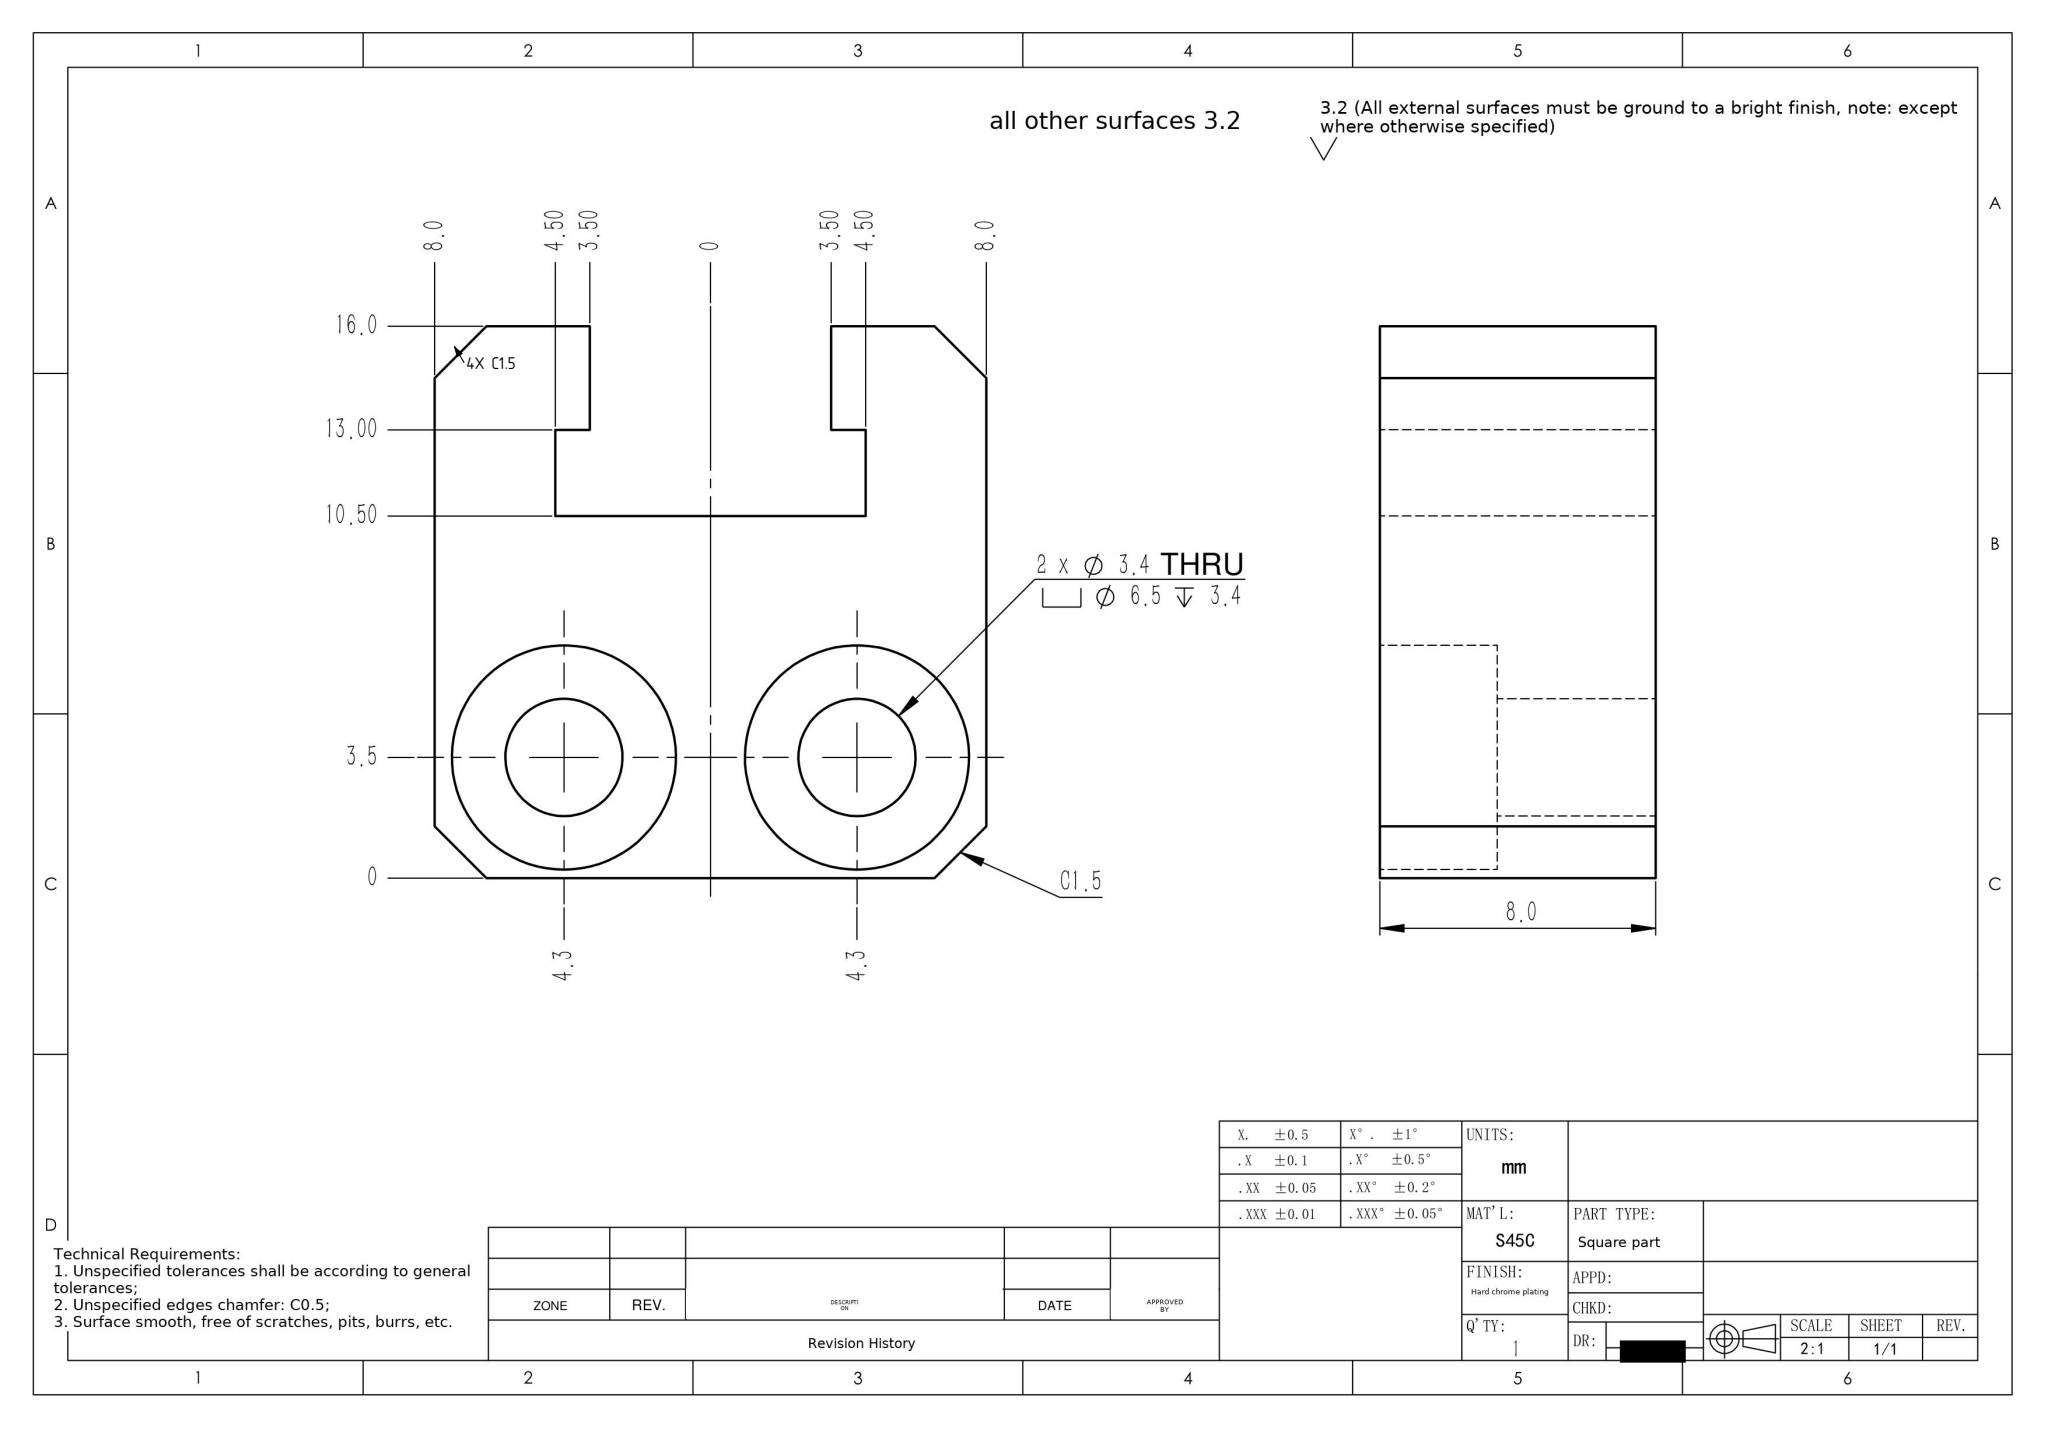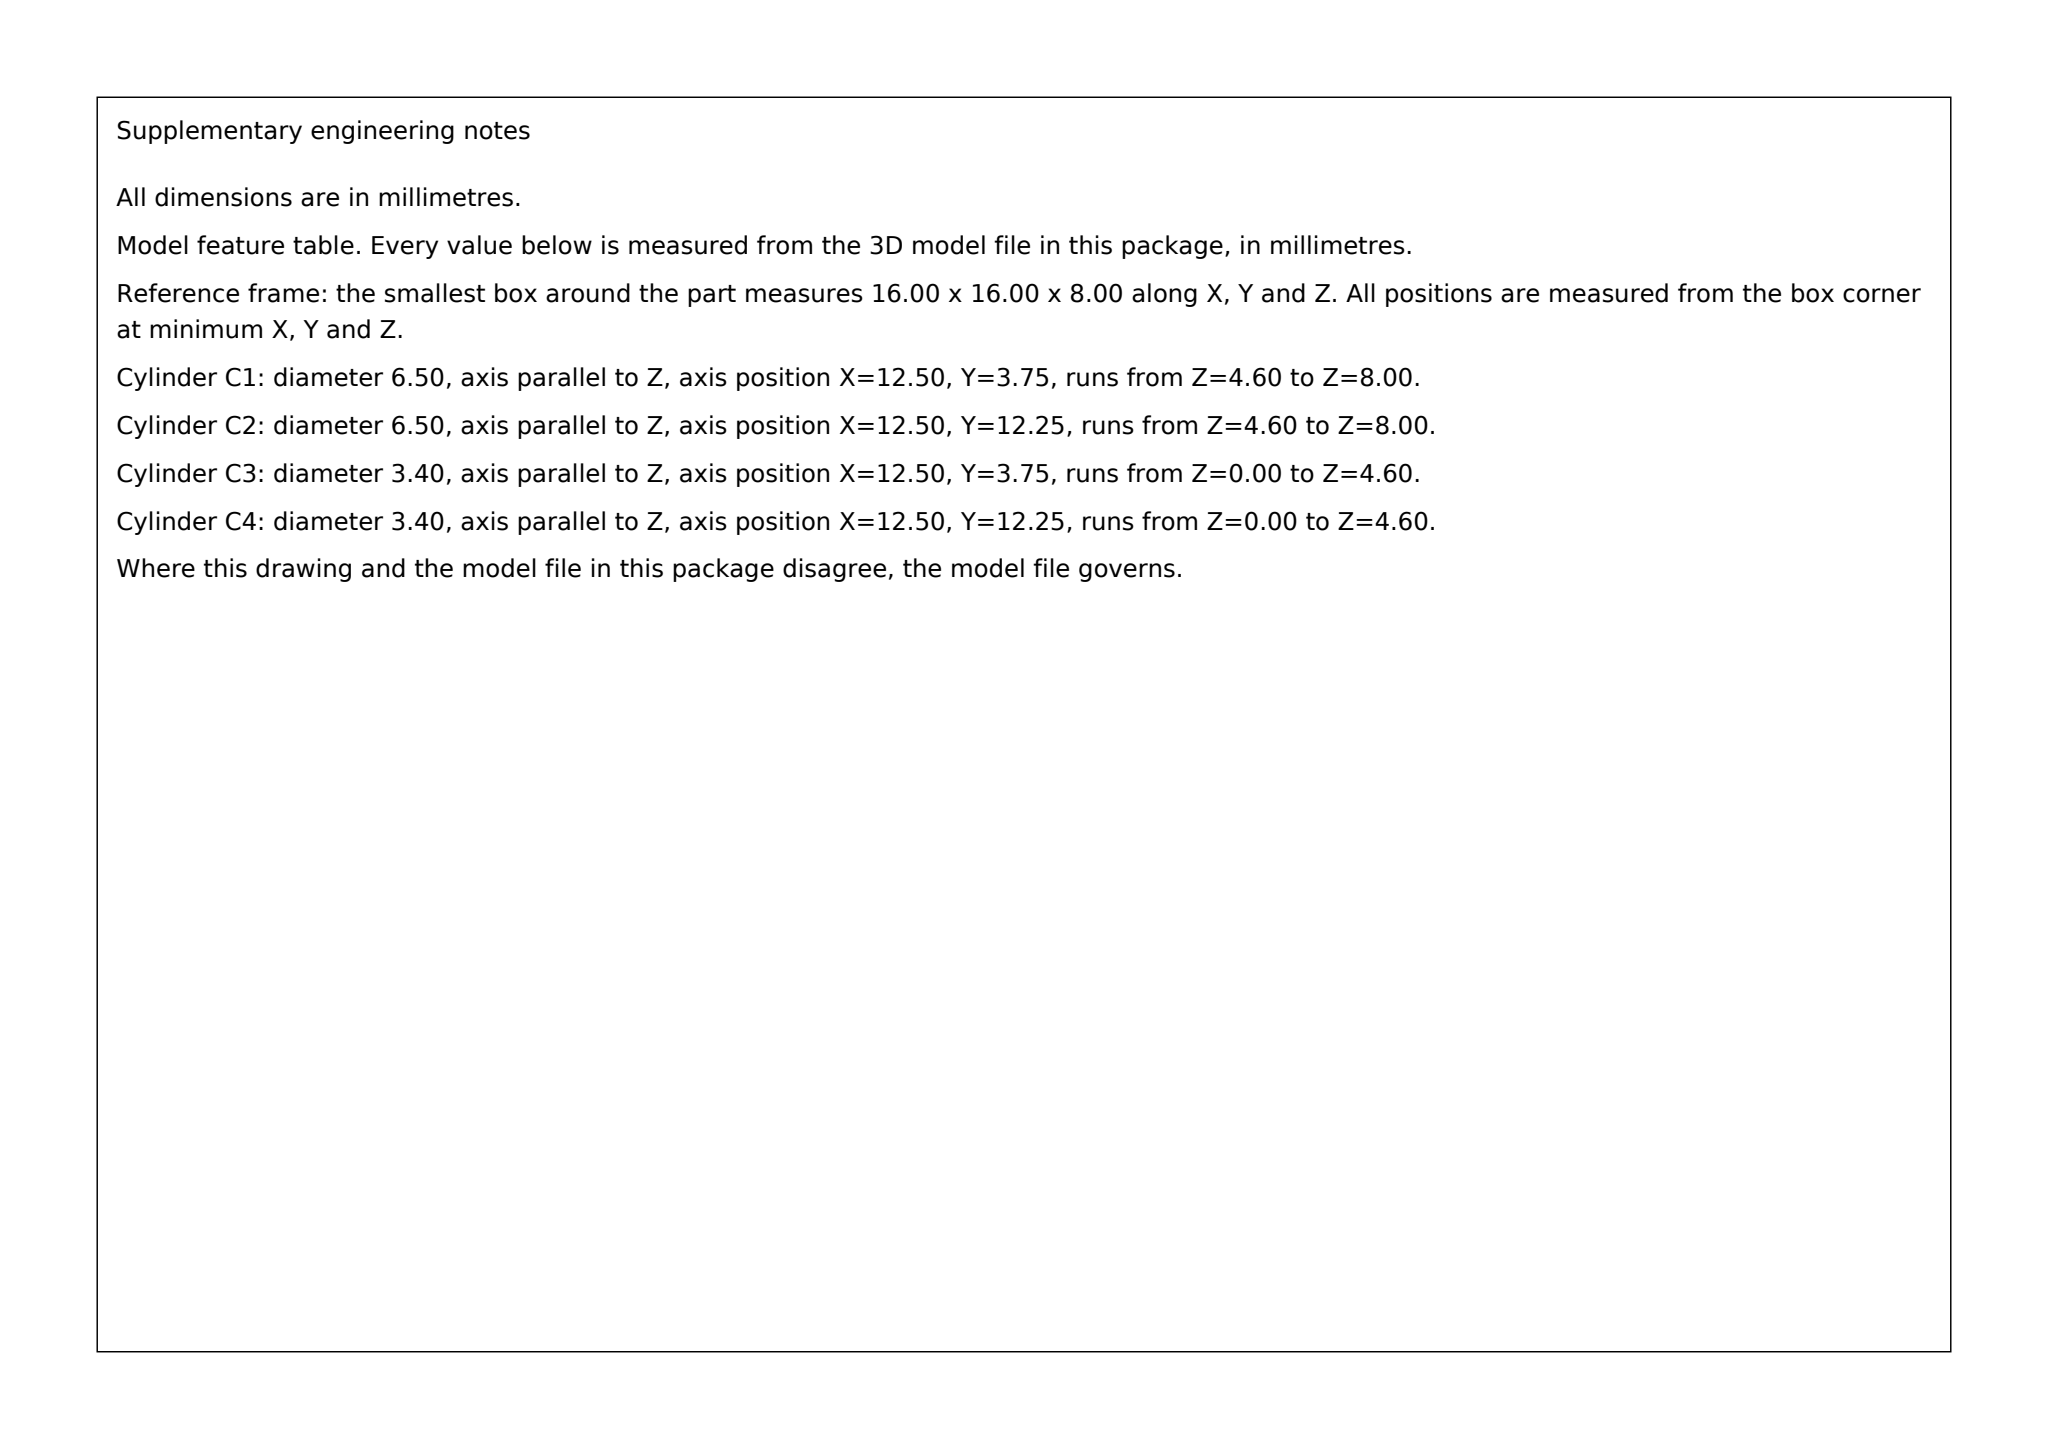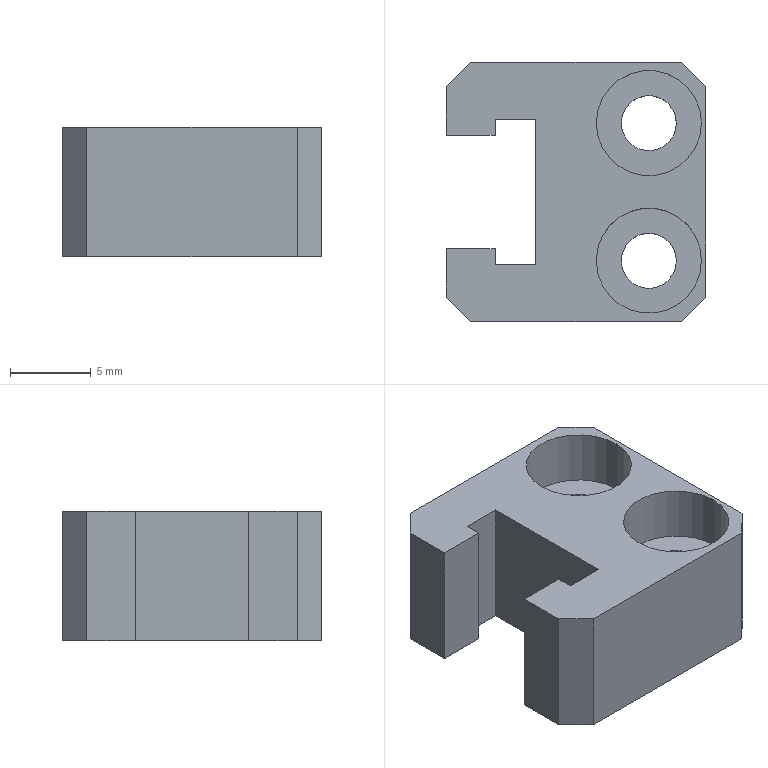Part | SolidWorks | mm | material S45C | 1 solid | 28 faces | box 16 x 16 x 8 mm | volume 1355 mm3 | plane 20 | cylinder 8 | commonest cylinder face diameters 6.5 x4 3.4 x4
Drawing notes:
4X C1.5 x 45° AT CORNERS OF 16 x 16 OUTLINE | from the solid: Bbox 16x16x8; outline bounded by planes x=0/16, y=0/16; all four outline corners broken equally, matching existing C1.5 callout (part symmetric about y=8 centerline)
build123d program:
from build123d import *

# Parameters (mm, degrees)
SKETCH1_W                                       = 16
SKETCH1_H                                       = 16
BOSS_EXTRUDE1_DEPTH                             = 8
M3_HEX_SOCKET_HEAD_CAP_SCREW_CBORE1_D           = 3.4
M3_HEX_SOCKET_HEAD_CAP_SCREW_CBORE1_CBORE_D     = 6.5
M3_HEX_SOCKET_HEAD_CAP_SCREW_CBORE1_CBORE_DEPTH = 3.4
CUT_EXTRUDE1_DEPTH                              = 20.596
CHAMFER1_SIZE                                   = 1.5


with BuildPart() as part:
    # Sketch1 → Boss-Extrude1 (new body)
    with BuildSketch(Plane.XY):
        with Locations((8, 0)):
            Rectangle(SKETCH1_W, SKETCH1_H)
    extrude(amount=BOSS_EXTRUDE1_DEPTH)

    # M3 Hex Socket Head Cap Screw CBORE1 (through all)
    with Locations(Plane.XY.offset(8)):
        with Locations((12.5, 4.25), (12.5, -4.25)):
            CounterBoreHole(M3_HEX_SOCKET_HEAD_CAP_SCREW_CBORE1_D / 2, M3_HEX_SOCKET_HEAD_CAP_SCREW_CBORE1_CBORE_D / 2, M3_HEX_SOCKET_HEAD_CAP_SCREW_CBORE1_CBORE_DEPTH)

    # Sketch4 → Cut-Extrude1 (cut, through all)
    with BuildSketch(Plane.XY.offset(8)):
        Polygon((0, -3.5), (0, 3.5), (3, 3.5), (3, 4.5), (5.5, 4.5), (5.5, -4.5), (3, -4.5), (3, -3.5), align=None)
    extrude(amount=-CUT_EXTRUDE1_DEPTH, mode=Mode.SUBTRACT)

    # Chamfer1
    chamfer1_edges = [part.edges().sort_by_distance(p)[0] for p in [
        (0, 8, 4),
        (16, 8, 4),
        (16, -8, 4),
        (0, -8, 4),
    ]]
    chamfer(chamfer1_edges, length=CHAMFER1_SIZE)


solid = part.part
STEP:
#1=CARTESIAN_POINT('',(9.25,4.25,4.6));
#2=VERTEX_POINT('',#1);
#3=CARTESIAN_POINT('',(15.75,4.25,4.6));
#4=VERTEX_POINT('',#3);
#5=CARTESIAN_POINT('',(12.5,4.25,4.6));
#6=DIRECTION('',(0.,0.,1.));
#7=DIRECTION('',(1.,0.,0.));
#8=AXIS2_PLACEMENT_3D('',#5,#6,#7);
#9=CIRCLE('',#8,3.25);
#10=EDGE_CURVE('',#2,#4,#9,.T.);
#11=ORIENTED_EDGE('',*,*,#10,.F.);
#12=CARTESIAN_POINT('',(9.25,4.25,8.));
#13=VERTEX_POINT('',#12);
#14=CARTESIAN_POINT('',(9.25,4.25,8.));
#15=DIRECTION('',(0.,0.,1.));
#16=VECTOR('',#15,1000.);
#17=LINE('',#14,#16);
#18=EDGE_CURVE('',#2,#13,#17,.T.);
#19=ORIENTED_EDGE('',*,*,#18,.T.);
#20=CARTESIAN_POINT('',(15.75,4.25,8.));
#21=VERTEX_POINT('',#20);
#22=CARTESIAN_POINT('',(12.5,4.25,8.));
#23=DIRECTION('',(0.,0.,1.));
#24=DIRECTION('',(1.,0.,0.));
#25=AXIS2_PLACEMENT_3D('',#22,#23,#24);
#26=CIRCLE('',#25,3.25);
#27=EDGE_CURVE('',#13,#21,#26,.T.);
#28=ORIENTED_EDGE('',*,*,#27,.T.);
#29=CARTESIAN_POINT('',(15.75,4.25,8.));
#30=DIRECTION('',(0.,0.,1.));
#31=VECTOR('',#30,1000.);
#32=LINE('',#29,#31);
#33=EDGE_CURVE('',#4,#21,#32,.T.);
#34=ORIENTED_EDGE('',*,*,#33,.F.);
#35=EDGE_LOOP('',(#11,#19,#28,#34));
#36=FACE_OUTER_BOUND('',#35,.T.);
#37=CARTESIAN_POINT('',(12.5,4.25,8.));
#38=DIRECTION('',(0.,0.,1.));
#39=DIRECTION('',(1.,0.,0.));
#40=AXIS2_PLACEMENT_3D('',#37,#38,#39);
#41=CYLINDRICAL_SURFACE('',#40,3.25);
#42=ADVANCED_FACE('',(#36),#41,.F.);
#43=CARTESIAN_POINT('',(10.8,4.25,0.));
#44=VERTEX_POINT('',#43);
#45=CARTESIAN_POINT('',(14.2,4.25,0.));
#46=VERTEX_POINT('',#45);
#47=CARTESIAN_POINT('',(12.5,4.25,0.));
#48=DIRECTION('',(0.,0.,1.));
#49=DIRECTION('',(1.,0.,0.));
#50=AXIS2_PLACEMENT_3D('',#47,#48,#49);
#51=CIRCLE('',#50,1.7);
#52=EDGE_CURVE('',#44,#46,#51,.T.);
#53=ORIENTED_EDGE('',*,*,#52,.F.);
#54=CARTESIAN_POINT('',(10.8,4.25,4.6));
#55=VERTEX_POINT('',#54);
#56=CARTESIAN_POINT('',(10.8,4.25,8.));
#57=DIRECTION('',(0.,0.,1.));
#58=VECTOR('',#57,1000.);
#59=LINE('',#56,#58);
#60=EDGE_CURVE('',#44,#55,#59,.T.);
#61=ORIENTED_EDGE('',*,*,#60,.T.);
#62=CARTESIAN_POINT('',(14.2,4.25,4.6));
#63=VERTEX_POINT('',#62);
#64=CARTESIAN_POINT('',(12.5,4.25,4.6));
#65=DIRECTION('',(0.,0.,1.));
#66=DIRECTION('',(1.,0.,0.));
#67=AXIS2_PLACEMENT_3D('',#64,#65,#66);
#68=CIRCLE('',#67,1.7);
#69=EDGE_CURVE('',#55,#63,#68,.T.);
#70=ORIENTED_EDGE('',*,*,#69,.T.);
#71=CARTESIAN_POINT('',(14.2,4.25,8.));
#72=DIRECTION('',(0.,0.,1.));
#73=VECTOR('',#72,1000.);
#74=LINE('',#71,#73);
#75=EDGE_CURVE('',#46,#63,#74,.T.);
#76=ORIENTED_EDGE('',*,*,#75,.F.);
#77=EDGE_LOOP('',(#53,#61,#70,#76));
#78=FACE_OUTER_BOUND('',#77,.T.);
#79=CARTESIAN_POINT('',(12.5,4.25,8.));
#80=DIRECTION('',(0.,0.,1.));
#81=DIRECTION('',(1.,0.,0.));
#82=AXIS2_PLACEMENT_3D('',#79,#80,#81);
#83=CYLINDRICAL_SURFACE('',#82,1.7);
#84=ADVANCED_FACE('',(#78),#83,.F.);
#85=CARTESIAN_POINT('',(9.25,-4.25,4.6));
#86=VERTEX_POINT('',#85);
#87=CARTESIAN_POINT('',(15.75,-4.25,4.6));
#88=VERTEX_POINT('',#87);
#89=CARTESIAN_POINT('',(12.5,-4.25,4.6));
#90=DIRECTION('',(0.,0.,1.));
#91=DIRECTION('',(1.,0.,0.));
#92=AXIS2_PLACEMENT_3D('',#89,#90,#91);
#93=CIRCLE('',#92,3.25);
#94=EDGE_CURVE('',#86,#88,#93,.T.);
#95=ORIENTED_EDGE('',*,*,#94,.F.);
#96=CARTESIAN_POINT('',(9.25,-4.25,8.));
#97=VERTEX_POINT('',#96);
#98=CARTESIAN_POINT('',(9.25,-4.25,8.));
#99=DIRECTION('',(0.,0.,1.));
#100=VECTOR('',#99,1000.);
#101=LINE('',#98,#100);
#102=EDGE_CURVE('',#86,#97,#101,.T.);
#103=ORIENTED_EDGE('',*,*,#102,.T.);
#104=CARTESIAN_POINT('',(15.75,-4.25,8.));
#105=VERTEX_POINT('',#104);
#106=CARTESIAN_POINT('',(12.5,-4.25,8.));
#107=DIRECTION('',(0.,0.,1.));
#108=DIRECTION('',(1.,0.,0.));
#109=AXIS2_PLACEMENT_3D('',#106,#107,#108);
#110=CIRCLE('',#109,3.25);
#111=EDGE_CURVE('',#97,#105,#110,.T.);
#112=ORIENTED_EDGE('',*,*,#111,.T.);
#113=CARTESIAN_POINT('',(15.75,-4.25,8.));
#114=DIRECTION('',(0.,0.,1.));
#115=VECTOR('',#114,1000.);
#116=LINE('',#113,#115);
#117=EDGE_CURVE('',#88,#105,#116,.T.);
#118=ORIENTED_EDGE('',*,*,#117,.F.);
#119=EDGE_LOOP('',(#95,#103,#112,#118));
#120=FACE_OUTER_BOUND('',#119,.T.);
#121=CARTESIAN_POINT('',(12.5,-4.25,8.));
#122=DIRECTION('',(0.,0.,1.));
#123=DIRECTION('',(1.,0.,0.));
#124=AXIS2_PLACEMENT_3D('',#121,#122,#123);
#125=CYLINDRICAL_SURFACE('',#124,3.25);
#126=ADVANCED_FACE('',(#120),#125,.F.);
#127=CARTESIAN_POINT('',(10.8,-4.25,0.));
#128=VERTEX_POINT('',#127);
#129=CARTESIAN_POINT('',(14.2,-4.25,0.));
#130=VERTEX_POINT('',#129);
#131=CARTESIAN_POINT('',(12.5,-4.25,0.));
#132=DIRECTION('',(0.,0.,1.));
#133=DIRECTION('',(1.,0.,0.));
#134=AXIS2_PLACEMENT_3D('',#131,#132,#133);
#135=CIRCLE('',#134,1.7);
#136=EDGE_CURVE('',#128,#130,#135,.T.);
#137=ORIENTED_EDGE('',*,*,#136,.F.);
#138=CARTESIAN_POINT('',(10.8,-4.25,4.6));
#139=VERTEX_POINT('',#138);
#140=CARTESIAN_POINT('',(10.8,-4.25,8.));
#141=DIRECTION('',(0.,0.,1.));
#142=VECTOR('',#141,1000.);
#143=LINE('',#140,#142);
#144=EDGE_CURVE('',#128,#139,#143,.T.);
#145=ORIENTED_EDGE('',*,*,#144,.T.);
#146=CARTESIAN_POINT('',(14.2,-4.25,4.6));
#147=VERTEX_POINT('',#146);
#148=CARTESIAN_POINT('',(12.5,-4.25,4.6));
#149=DIRECTION('',(0.,0.,1.));
#150=DIRECTION('',(1.,0.,0.));
#151=AXIS2_PLACEMENT_3D('',#148,#149,#150);
#152=CIRCLE('',#151,1.7);
#153=EDGE_CURVE('',#139,#147,#152,.T.);
#154=ORIENTED_EDGE('',*,*,#153,.T.);
#155=CARTESIAN_POINT('',(14.2,-4.25,8.));
#156=DIRECTION('',(0.,0.,1.));
#157=VECTOR('',#156,1000.);
#158=LINE('',#155,#157);
#159=EDGE_CURVE('',#130,#147,#158,.T.);
#160=ORIENTED_EDGE('',*,*,#159,.F.);
#161=EDGE_LOOP('',(#137,#145,#154,#160));
#162=FACE_OUTER_BOUND('',#161,.T.);
#163=CARTESIAN_POINT('',(12.5,-4.25,8.));
#164=DIRECTION('',(0.,0.,1.));
#165=DIRECTION('',(1.,0.,0.));
#166=AXIS2_PLACEMENT_3D('',#163,#164,#165);
#167=CYLINDRICAL_SURFACE('',#166,1.7);
#168=ADVANCED_FACE('',(#162),#167,.F.);
#169=CARTESIAN_POINT('',(0.,-3.5,0.));
#170=VERTEX_POINT('',#169);
#171=CARTESIAN_POINT('',(0.,-6.5,0.));
#172=VERTEX_POINT('',#171);
#173=CARTESIAN_POINT('',(0.,8.,0.));
#174=DIRECTION('',(-0.,-1.,0.));
#175=VECTOR('',#174,1000.);
#176=LINE('',#173,#175);
#177=EDGE_CURVE('',#170,#172,#176,.T.);
#178=ORIENTED_EDGE('',*,*,#177,.T.);
#179=CARTESIAN_POINT('',(0.,-6.5,8.));
#180=VERTEX_POINT('',#179);
#181=CARTESIAN_POINT('',(0.,-6.5,8.));
#182=DIRECTION('',(0.,0.,1.));
#183=VECTOR('',#182,1000.);
#184=LINE('',#181,#183);
#185=EDGE_CURVE('',#172,#180,#184,.T.);
#186=ORIENTED_EDGE('',*,*,#185,.T.);
#187=CARTESIAN_POINT('',(0.,-3.5,8.));
#188=VERTEX_POINT('',#187);
#189=CARTESIAN_POINT('',(0.,8.,8.));
#190=DIRECTION('',(-0.,-1.,0.));
#191=VECTOR('',#190,1000.);
#192=LINE('',#189,#191);
#193=EDGE_CURVE('',#188,#180,#192,.T.);
#194=ORIENTED_EDGE('',*,*,#193,.F.);
#195=CARTESIAN_POINT('',(0.,-3.5,0.));
#196=DIRECTION('',(0.,0.,1.));
#197=VECTOR('',#196,1000.);
#198=LINE('',#195,#197);
#199=EDGE_CURVE('',#170,#188,#198,.T.);
#200=ORIENTED_EDGE('',*,*,#199,.F.);
#201=EDGE_LOOP('',(#178,#186,#194,#200));
#202=FACE_OUTER_BOUND('',#201,.T.);
#203=CARTESIAN_POINT('',(0.,8.,8.));
#204=DIRECTION('',(1.,-0.,0.));
#205=DIRECTION('',(0.,1.,0.));
#206=AXIS2_PLACEMENT_3D('',#203,#204,#205);
#207=PLANE('',#206);
#208=ADVANCED_FACE('',(#202),#207,.F.);
#209=CARTESIAN_POINT('',(0.,6.5,8.));
#210=VERTEX_POINT('',#209);
#211=CARTESIAN_POINT('',(0.,3.5,8.));
#212=VERTEX_POINT('',#211);
#213=CARTESIAN_POINT('',(0.,8.,8.));
#214=DIRECTION('',(-0.,-1.,0.));
#215=VECTOR('',#214,1000.);
#216=LINE('',#213,#215);
#217=EDGE_CURVE('',#210,#212,#216,.T.);
#218=ORIENTED_EDGE('',*,*,#217,.F.);
#219=CARTESIAN_POINT('',(0.,6.5,0.));
#220=VERTEX_POINT('',#219);
#221=CARTESIAN_POINT('',(0.,6.5,8.));
#222=DIRECTION('',(0.,0.,-1.));
#223=VECTOR('',#222,1000.);
#224=LINE('',#221,#223);
#225=EDGE_CURVE('',#210,#220,#224,.T.);
#226=ORIENTED_EDGE('',*,*,#225,.T.);
#227=CARTESIAN_POINT('',(0.,3.5,0.));
#228=VERTEX_POINT('',#227);
#229=CARTESIAN_POINT('',(0.,8.,0.));
#230=DIRECTION('',(-0.,-1.,0.));
#231=VECTOR('',#230,1000.);
#232=LINE('',#229,#231);
#233=EDGE_CURVE('',#220,#228,#232,.T.);
#234=ORIENTED_EDGE('',*,*,#233,.T.);
#235=CARTESIAN_POINT('',(0.,3.5,0.));
#236=DIRECTION('',(0.,0.,1.));
#237=VECTOR('',#236,1000.);
#238=LINE('',#235,#237);
#239=EDGE_CURVE('',#228,#212,#238,.T.);
#240=ORIENTED_EDGE('',*,*,#239,.T.);
#241=EDGE_LOOP('',(#218,#226,#234,#240));
#242=FACE_OUTER_BOUND('',#241,.T.);
#243=CARTESIAN_POINT('',(0.,8.,8.));
#244=DIRECTION('',(1.,-0.,0.));
#245=DIRECTION('',(0.,1.,0.));
#246=AXIS2_PLACEMENT_3D('',#243,#244,#245);
#247=PLANE('',#246);
#248=ADVANCED_FACE('',(#242),#247,.F.);
#249=CARTESIAN_POINT('',(1.5,-8.,0.));
#250=VERTEX_POINT('',#249);
#251=CARTESIAN_POINT('',(14.5,-8.,0.));
#252=VERTEX_POINT('',#251);
#253=CARTESIAN_POINT('',(0.,-8.,0.));
#254=DIRECTION('',(1.,0.,0.));
#255=VECTOR('',#254,1000.);
#256=LINE('',#253,#255);
#257=EDGE_CURVE('',#250,#252,#256,.T.);
#258=ORIENTED_EDGE('',*,*,#257,.T.);
#259=CARTESIAN_POINT('',(14.5,-8.,8.));
#260=VERTEX_POINT('',#259);
#261=CARTESIAN_POINT('',(14.5,-8.,8.));
#262=DIRECTION('',(0.,0.,1.));
#263=VECTOR('',#262,1000.);
#264=LINE('',#261,#263);
#265=EDGE_CURVE('',#252,#260,#264,.T.);
#266=ORIENTED_EDGE('',*,*,#265,.T.);
#267=CARTESIAN_POINT('',(1.5,-8.,8.));
#268=VERTEX_POINT('',#267);
#269=CARTESIAN_POINT('',(0.,-8.,8.));
#270=DIRECTION('',(1.,0.,0.));
#271=VECTOR('',#270,1000.);
#272=LINE('',#269,#271);
#273=EDGE_CURVE('',#268,#260,#272,.T.);
#274=ORIENTED_EDGE('',*,*,#273,.F.);
#275=CARTESIAN_POINT('',(1.5,-8.,8.));
#276=DIRECTION('',(0.,0.,-1.));
#277=VECTOR('',#276,1000.);
#278=LINE('',#275,#277);
#279=EDGE_CURVE('',#268,#250,#278,.T.);
#280=ORIENTED_EDGE('',*,*,#279,.T.);
#281=EDGE_LOOP('',(#258,#266,#274,#280));
#282=FACE_OUTER_BOUND('',#281,.T.);
#283=CARTESIAN_POINT('',(0.,-8.,8.));
#284=DIRECTION('',(0.,1.,0.));
#285=DIRECTION('',(0.,0.,1.));
#286=AXIS2_PLACEMENT_3D('',#283,#284,#285);
#287=PLANE('',#286);
#288=ADVANCED_FACE('',(#282),#287,.F.);
#289=CARTESIAN_POINT('',(16.,-6.5,0.));
#290=VERTEX_POINT('',#289);
#291=CARTESIAN_POINT('',(16.,6.5,0.));
#292=VERTEX_POINT('',#291);
#293=CARTESIAN_POINT('',(16.,8.,0.));
#294=DIRECTION('',(0.,1.,0.));
#295=VECTOR('',#294,1000.);
#296=LINE('',#293,#295);
#297=EDGE_CURVE('',#290,#292,#296,.T.);
#298=ORIENTED_EDGE('',*,*,#297,.T.);
#299=CARTESIAN_POINT('',(16.,6.5,8.));
#300=VERTEX_POINT('',#299);
#301=CARTESIAN_POINT('',(16.,6.5,8.));
#302=DIRECTION('',(0.,0.,1.));
#303=VECTOR('',#302,1000.);
#304=LINE('',#301,#303);
#305=EDGE_CURVE('',#292,#300,#304,.T.);
#306=ORIENTED_EDGE('',*,*,#305,.T.);
#307=CARTESIAN_POINT('',(16.,-6.5,8.));
#308=VERTEX_POINT('',#307);
#309=CARTESIAN_POINT('',(16.,8.,8.));
#310=DIRECTION('',(0.,1.,0.));
#311=VECTOR('',#310,1000.);
#312=LINE('',#309,#311);
#313=EDGE_CURVE('',#308,#300,#312,.T.);
#314=ORIENTED_EDGE('',*,*,#313,.F.);
#315=CARTESIAN_POINT('',(16.,-6.5,8.));
#316=DIRECTION('',(0.,0.,-1.));
#317=VECTOR('',#316,1000.);
#318=LINE('',#315,#317);
#319=EDGE_CURVE('',#308,#290,#318,.T.);
#320=ORIENTED_EDGE('',*,*,#319,.T.);
#321=EDGE_LOOP('',(#298,#306,#314,#320));
#322=FACE_OUTER_BOUND('',#321,.T.);
#323=CARTESIAN_POINT('',(16.,8.,8.));
#324=DIRECTION('',(-1.,0.,0.));
#325=DIRECTION('',(0.,0.,1.));
#326=AXIS2_PLACEMENT_3D('',#323,#324,#325);
#327=PLANE('',#326);
#328=ADVANCED_FACE('',(#322),#327,.F.);
#329=CARTESIAN_POINT('',(14.5,8.,8.));
#330=VERTEX_POINT('',#329);
#331=CARTESIAN_POINT('',(1.5,8.,8.));
#332=VERTEX_POINT('',#331);
#333=CARTESIAN_POINT('',(0.,8.,8.));
#334=DIRECTION('',(-1.,0.,0.));
#335=VECTOR('',#334,1000.);
#336=LINE('',#333,#335);
#337=EDGE_CURVE('',#330,#332,#336,.T.);
#338=ORIENTED_EDGE('',*,*,#337,.F.);
#339=CARTESIAN_POINT('',(14.5,8.,0.));
#340=VERTEX_POINT('',#339);
#341=CARTESIAN_POINT('',(14.5,8.,8.));
#342=DIRECTION('',(0.,0.,-1.));
#343=VECTOR('',#342,1000.);
#344=LINE('',#341,#343);
#345=EDGE_CURVE('',#330,#340,#344,.T.);
#346=ORIENTED_EDGE('',*,*,#345,.T.);
#347=CARTESIAN_POINT('',(1.5,8.,0.));
#348=VERTEX_POINT('',#347);
#349=CARTESIAN_POINT('',(0.,8.,0.));
#350=DIRECTION('',(-1.,0.,0.));
#351=VECTOR('',#350,1000.);
#352=LINE('',#349,#351);
#353=EDGE_CURVE('',#340,#348,#352,.T.);
#354=ORIENTED_EDGE('',*,*,#353,.T.);
#355=CARTESIAN_POINT('',(1.5,8.,8.));
#356=DIRECTION('',(0.,0.,1.));
#357=VECTOR('',#356,1000.);
#358=LINE('',#355,#357);
#359=EDGE_CURVE('',#348,#332,#358,.T.);
#360=ORIENTED_EDGE('',*,*,#359,.T.);
#361=EDGE_LOOP('',(#338,#346,#354,#360));
#362=FACE_OUTER_BOUND('',#361,.T.);
#363=CARTESIAN_POINT('',(0.,8.,8.));
#364=DIRECTION('',(0.,-1.,0.));
#365=DIRECTION('',(0.,0.,-1.));
#366=AXIS2_PLACEMENT_3D('',#363,#364,#365);
#367=PLANE('',#366);
#368=ADVANCED_FACE('',(#362),#367,.F.);
#369=ORIENTED_EDGE('',*,*,#313,.T.);
#370=CARTESIAN_POINT('',(11.25,11.25,8.));
#371=DIRECTION('',(-0.7071,0.7071,0.));
#372=VECTOR('',#371,1000.);
#373=LINE('',#370,#372);
#374=EDGE_CURVE('',#300,#330,#373,.T.);
#375=ORIENTED_EDGE('',*,*,#374,.T.);
#376=ORIENTED_EDGE('',*,*,#337,.T.);
#377=CARTESIAN_POINT('',(-3.25,3.25,8.));
#378=DIRECTION('',(-0.7071,-0.7071,0.));
#379=VECTOR('',#378,1000.);
#380=LINE('',#377,#379);
#381=EDGE_CURVE('',#332,#210,#380,.T.);
#382=ORIENTED_EDGE('',*,*,#381,.T.);
#383=ORIENTED_EDGE('',*,*,#217,.T.);
#384=CARTESIAN_POINT('',(3.,3.5,8.));
#385=VERTEX_POINT('',#384);
#386=CARTESIAN_POINT('',(0.,3.5,8.));
#387=DIRECTION('',(-1.,0.,0.));
#388=VECTOR('',#387,1000.);
#389=LINE('',#386,#388);
#390=EDGE_CURVE('',#385,#212,#389,.T.);
#391=ORIENTED_EDGE('',*,*,#390,.F.);
#392=CARTESIAN_POINT('',(3.,4.5,8.));
#393=VERTEX_POINT('',#392);
#394=CARTESIAN_POINT('',(3.,3.5,8.));
#395=DIRECTION('',(-0.,-1.,0.));
#396=VECTOR('',#395,1000.);
#397=LINE('',#394,#396);
#398=EDGE_CURVE('',#393,#385,#397,.T.);
#399=ORIENTED_EDGE('',*,*,#398,.F.);
#400=CARTESIAN_POINT('',(5.5,4.5,8.));
#401=VERTEX_POINT('',#400);
#402=CARTESIAN_POINT('',(3.,4.5,8.));
#403=DIRECTION('',(-1.,0.,0.));
#404=VECTOR('',#403,1000.);
#405=LINE('',#402,#404);
#406=EDGE_CURVE('',#401,#393,#405,.T.);
#407=ORIENTED_EDGE('',*,*,#406,.F.);
#408=CARTESIAN_POINT('',(5.5,-4.5,8.));
#409=VERTEX_POINT('',#408);
#410=CARTESIAN_POINT('',(5.5,4.5,8.));
#411=DIRECTION('',(0.,1.,0.));
#412=VECTOR('',#411,1000.);
#413=LINE('',#410,#412);
#414=EDGE_CURVE('',#409,#401,#413,.T.);
#415=ORIENTED_EDGE('',*,*,#414,.F.);
#416=CARTESIAN_POINT('',(3.,-4.5,8.));
#417=VERTEX_POINT('',#416);
#418=CARTESIAN_POINT('',(5.5,-4.5,8.));
#419=DIRECTION('',(1.,0.,0.));
#420=VECTOR('',#419,1000.);
#421=LINE('',#418,#420);
#422=EDGE_CURVE('',#417,#409,#421,.T.);
#423=ORIENTED_EDGE('',*,*,#422,.F.);
#424=CARTESIAN_POINT('',(3.,-3.5,8.));
#425=VERTEX_POINT('',#424);
#426=CARTESIAN_POINT('',(3.,-4.5,8.));
#427=DIRECTION('',(0.,-1.,0.));
#428=VECTOR('',#427,1000.);
#429=LINE('',#426,#428);
#430=EDGE_CURVE('',#425,#417,#429,.T.);
#431=ORIENTED_EDGE('',*,*,#430,.F.);
#432=CARTESIAN_POINT('',(3.,-3.5,8.));
#433=DIRECTION('',(1.,0.,0.));
#434=VECTOR('',#433,1000.);
#435=LINE('',#432,#434);
#436=EDGE_CURVE('',#188,#425,#435,.T.);
#437=ORIENTED_EDGE('',*,*,#436,.F.);
#438=ORIENTED_EDGE('',*,*,#193,.T.);
#439=CARTESIAN_POINT('',(-3.25,-3.25,8.));
#440=DIRECTION('',(0.7071,-0.7071,0.));
#441=VECTOR('',#440,1000.);
#442=LINE('',#439,#441);
#443=EDGE_CURVE('',#180,#268,#442,.T.);
#444=ORIENTED_EDGE('',*,*,#443,.T.);
#445=ORIENTED_EDGE('',*,*,#273,.T.);
#446=CARTESIAN_POINT('',(11.25,-11.25,8.));
#447=DIRECTION('',(0.7071,0.7071,0.));
#448=VECTOR('',#447,1000.);
#449=LINE('',#446,#448);
#450=EDGE_CURVE('',#260,#308,#449,.T.);
#451=ORIENTED_EDGE('',*,*,#450,.T.);
#452=EDGE_LOOP('',(#369,#375,#376,#382,#383,#391,#399,#407,#415,#423,#431,#437,#438,#444,#445,#451));
#453=FACE_OUTER_BOUND('',#452,.T.);
#454=CARTESIAN_POINT('',(12.5,4.25,8.));
#455=DIRECTION('',(0.,0.,1.));
#456=DIRECTION('',(1.,0.,0.));
#457=AXIS2_PLACEMENT_3D('',#454,#455,#456);
#458=CIRCLE('',#457,3.25);
#459=EDGE_CURVE('',#21,#13,#458,.T.);
#460=ORIENTED_EDGE('',*,*,#459,.F.);
#461=ORIENTED_EDGE('',*,*,#27,.F.);
#462=EDGE_LOOP('',(#460,#461));
#463=FACE_BOUND('',#462,.T.);
#464=CARTESIAN_POINT('',(12.5,-4.25,8.));
#465=DIRECTION('',(0.,0.,1.));
#466=DIRECTION('',(1.,0.,0.));
#467=AXIS2_PLACEMENT_3D('',#464,#465,#466);
#468=CIRCLE('',#467,3.25);
#469=EDGE_CURVE('',#105,#97,#468,.T.);
#470=ORIENTED_EDGE('',*,*,#469,.F.);
#471=ORIENTED_EDGE('',*,*,#111,.F.);
#472=EDGE_LOOP('',(#470,#471));
#473=FACE_BOUND('',#472,.T.);
#474=CARTESIAN_POINT('',(0.,0.,8.));
#475=DIRECTION('',(0.,0.,1.));
#476=DIRECTION('',(1.,0.,0.));
#477=AXIS2_PLACEMENT_3D('',#474,#475,#476);
#478=PLANE('',#477);
#479=ADVANCED_FACE('',(#453,#463,#473),#478,.T.);
#480=ORIENTED_EDGE('',*,*,#353,.F.);
#481=CARTESIAN_POINT('',(14.5,8.,0.));
#482=DIRECTION('',(0.7071,-0.7071,0.));
#483=VECTOR('',#482,1000.);
#484=LINE('',#481,#483);
#485=EDGE_CURVE('',#340,#292,#484,.T.);
#486=ORIENTED_EDGE('',*,*,#485,.T.);
#487=ORIENTED_EDGE('',*,*,#297,.F.);
#488=CARTESIAN_POINT('',(16.,-6.5,0.));
#489=DIRECTION('',(-0.7071,-0.7071,0.));
#490=VECTOR('',#489,1000.);
#491=LINE('',#488,#490);
#492=EDGE_CURVE('',#290,#252,#491,.T.);
#493=ORIENTED_EDGE('',*,*,#492,.T.);
#494=ORIENTED_EDGE('',*,*,#257,.F.);
#495=CARTESIAN_POINT('',(1.5,-8.,0.));
#496=DIRECTION('',(-0.7071,0.7071,0.));
#497=VECTOR('',#496,1000.);
#498=LINE('',#495,#497);
#499=EDGE_CURVE('',#250,#172,#498,.T.);
#500=ORIENTED_EDGE('',*,*,#499,.T.);
#501=ORIENTED_EDGE('',*,*,#177,.F.);
#502=CARTESIAN_POINT('',(3.,-3.5,0.));
#503=VERTEX_POINT('',#502);
#504=CARTESIAN_POINT('',(3.,-3.5,0.));
#505=DIRECTION('',(1.,0.,0.));
#506=VECTOR('',#505,1000.);
#507=LINE('',#504,#506);
#508=EDGE_CURVE('',#170,#503,#507,.T.);
#509=ORIENTED_EDGE('',*,*,#508,.T.);
#510=CARTESIAN_POINT('',(3.,-4.5,0.));
#511=VERTEX_POINT('',#510);
#512=CARTESIAN_POINT('',(3.,-4.5,0.));
#513=DIRECTION('',(0.,-1.,0.));
#514=VECTOR('',#513,1000.);
#515=LINE('',#512,#514);
#516=EDGE_CURVE('',#503,#511,#515,.T.);
#517=ORIENTED_EDGE('',*,*,#516,.T.);
#518=CARTESIAN_POINT('',(5.5,-4.5,0.));
#519=VERTEX_POINT('',#518);
#520=CARTESIAN_POINT('',(5.5,-4.5,0.));
#521=DIRECTION('',(1.,0.,0.));
#522=VECTOR('',#521,1000.);
#523=LINE('',#520,#522);
#524=EDGE_CURVE('',#511,#519,#523,.T.);
#525=ORIENTED_EDGE('',*,*,#524,.T.);
#526=CARTESIAN_POINT('',(5.5,4.5,0.));
#527=VERTEX_POINT('',#526);
#528=CARTESIAN_POINT('',(5.5,4.5,0.));
#529=DIRECTION('',(0.,1.,0.));
#530=VECTOR('',#529,1000.);
#531=LINE('',#528,#530);
#532=EDGE_CURVE('',#519,#527,#531,.T.);
#533=ORIENTED_EDGE('',*,*,#532,.T.);
#534=CARTESIAN_POINT('',(3.,4.5,0.));
#535=VERTEX_POINT('',#534);
#536=CARTESIAN_POINT('',(3.,4.5,0.));
#537=DIRECTION('',(-1.,0.,0.));
#538=VECTOR('',#537,1000.);
#539=LINE('',#536,#538);
#540=EDGE_CURVE('',#527,#535,#539,.T.);
#541=ORIENTED_EDGE('',*,*,#540,.T.);
#542=CARTESIAN_POINT('',(3.,3.5,0.));
#543=VERTEX_POINT('',#542);
#544=CARTESIAN_POINT('',(3.,3.5,0.));
#545=DIRECTION('',(-0.,-1.,0.));
#546=VECTOR('',#545,1000.);
#547=LINE('',#544,#546);
#548=EDGE_CURVE('',#535,#543,#547,.T.);
#549=ORIENTED_EDGE('',*,*,#548,.T.);
#550=CARTESIAN_POINT('',(0.,3.5,0.));
#551=DIRECTION('',(-1.,0.,0.));
#552=VECTOR('',#551,1000.);
#553=LINE('',#550,#552);
#554=EDGE_CURVE('',#543,#228,#553,.T.);
#555=ORIENTED_EDGE('',*,*,#554,.T.);
#556=ORIENTED_EDGE('',*,*,#233,.F.);
#557=CARTESIAN_POINT('',(0.,6.5,0.));
#558=DIRECTION('',(0.7071,0.7071,0.));
#559=VECTOR('',#558,1000.);
#560=LINE('',#557,#559);
#561=EDGE_CURVE('',#220,#348,#560,.T.);
#562=ORIENTED_EDGE('',*,*,#561,.T.);
#563=EDGE_LOOP('',(#480,#486,#487,#493,#494,#500,#501,#509,#517,#525,#533,#541,#549,#555,#556,#562));
#564=FACE_OUTER_BOUND('',#563,.T.);
#565=CARTESIAN_POINT('',(12.5,4.25,0.));
#566=DIRECTION('',(0.,0.,1.));
#567=DIRECTION('',(1.,0.,0.));
#568=AXIS2_PLACEMENT_3D('',#565,#566,#567);
#569=CIRCLE('',#568,1.7);
#570=EDGE_CURVE('',#46,#44,#569,.T.);
#571=ORIENTED_EDGE('',*,*,#570,.T.);
#572=ORIENTED_EDGE('',*,*,#52,.T.);
#573=EDGE_LOOP('',(#571,#572));
#574=FACE_BOUND('',#573,.T.);
#575=CARTESIAN_POINT('',(12.5,-4.25,0.));
#576=DIRECTION('',(0.,0.,1.));
#577=DIRECTION('',(1.,0.,0.));
#578=AXIS2_PLACEMENT_3D('',#575,#576,#577);
#579=CIRCLE('',#578,1.7);
#580=EDGE_CURVE('',#130,#128,#579,.T.);
#581=ORIENTED_EDGE('',*,*,#580,.T.);
#582=ORIENTED_EDGE('',*,*,#136,.T.);
#583=EDGE_LOOP('',(#581,#582));
#584=FACE_BOUND('',#583,.T.);
#585=CARTESIAN_POINT('',(0.,0.,0.));
#586=DIRECTION('',(0.,0.,1.));
#587=DIRECTION('',(1.,0.,0.));
#588=AXIS2_PLACEMENT_3D('',#585,#586,#587);
#589=PLANE('',#588);
#590=ADVANCED_FACE('',(#564,#574,#584),#589,.F.);
#591=ORIENTED_EDGE('',*,*,#144,.F.);
#592=ORIENTED_EDGE('',*,*,#580,.F.);
#593=ORIENTED_EDGE('',*,*,#159,.T.);
#594=CARTESIAN_POINT('',(12.5,-4.25,4.6));
#595=DIRECTION('',(0.,0.,1.));
#596=DIRECTION('',(1.,0.,0.));
#597=AXIS2_PLACEMENT_3D('',#594,#595,#596);
#598=CIRCLE('',#597,1.7);
#599=EDGE_CURVE('',#147,#139,#598,.T.);
#600=ORIENTED_EDGE('',*,*,#599,.T.);
#601=EDGE_LOOP('',(#591,#592,#593,#600));
#602=FACE_OUTER_BOUND('',#601,.T.);
#603=CARTESIAN_POINT('',(12.5,-4.25,8.));
#604=DIRECTION('',(0.,0.,1.));
#605=DIRECTION('',(1.,0.,0.));
#606=AXIS2_PLACEMENT_3D('',#603,#604,#605);
#607=CYLINDRICAL_SURFACE('',#606,1.7);
#608=ADVANCED_FACE('',(#602),#607,.F.);
#609=ORIENTED_EDGE('',*,*,#599,.F.);
#610=ORIENTED_EDGE('',*,*,#153,.F.);
#611=EDGE_LOOP('',(#609,#610));
#612=FACE_BOUND('',#611,.T.);
#613=CARTESIAN_POINT('',(12.5,-4.25,4.6));
#614=DIRECTION('',(0.,0.,1.));
#615=DIRECTION('',(1.,0.,0.));
#616=AXIS2_PLACEMENT_3D('',#613,#614,#615);
#617=CIRCLE('',#616,3.25);
#618=EDGE_CURVE('',#88,#86,#617,.T.);
#619=ORIENTED_EDGE('',*,*,#618,.T.);
#620=ORIENTED_EDGE('',*,*,#94,.T.);
#621=EDGE_LOOP('',(#619,#620));
#622=FACE_OUTER_BOUND('',#621,.T.);
#623=CARTESIAN_POINT('',(14.2,-4.25,4.6));
#624=DIRECTION('',(0.,0.,-1.));
#625=DIRECTION('',(-1.,0.,0.));
#626=AXIS2_PLACEMENT_3D('',#623,#624,#625);
#627=PLANE('',#626);
#628=ADVANCED_FACE('',(#612,#622),#627,.F.);
#629=ORIENTED_EDGE('',*,*,#102,.F.);
#630=ORIENTED_EDGE('',*,*,#618,.F.);
#631=ORIENTED_EDGE('',*,*,#117,.T.);
#632=ORIENTED_EDGE('',*,*,#469,.T.);
#633=EDGE_LOOP('',(#629,#630,#631,#632));
#634=FACE_OUTER_BOUND('',#633,.T.);
#635=CARTESIAN_POINT('',(12.5,-4.25,8.));
#636=DIRECTION('',(0.,0.,1.));
#637=DIRECTION('',(1.,0.,0.));
#638=AXIS2_PLACEMENT_3D('',#635,#636,#637);
#639=CYLINDRICAL_SURFACE('',#638,3.25);
#640=ADVANCED_FACE('',(#634),#639,.F.);
#641=ORIENTED_EDGE('',*,*,#60,.F.);
#642=ORIENTED_EDGE('',*,*,#570,.F.);
#643=ORIENTED_EDGE('',*,*,#75,.T.);
#644=CARTESIAN_POINT('',(12.5,4.25,4.6));
#645=DIRECTION('',(0.,0.,1.));
#646=DIRECTION('',(1.,0.,0.));
#647=AXIS2_PLACEMENT_3D('',#644,#645,#646);
#648=CIRCLE('',#647,1.7);
#649=EDGE_CURVE('',#63,#55,#648,.T.);
#650=ORIENTED_EDGE('',*,*,#649,.T.);
#651=EDGE_LOOP('',(#641,#642,#643,#650));
#652=FACE_OUTER_BOUND('',#651,.T.);
#653=CARTESIAN_POINT('',(12.5,4.25,8.));
#654=DIRECTION('',(0.,0.,1.));
#655=DIRECTION('',(1.,0.,0.));
#656=AXIS2_PLACEMENT_3D('',#653,#654,#655);
#657=CYLINDRICAL_SURFACE('',#656,1.7);
#658=ADVANCED_FACE('',(#652),#657,.F.);
#659=ORIENTED_EDGE('',*,*,#649,.F.);
#660=ORIENTED_EDGE('',*,*,#69,.F.);
#661=EDGE_LOOP('',(#659,#660));
#662=FACE_BOUND('',#661,.T.);
#663=CARTESIAN_POINT('',(12.5,4.25,4.6));
#664=DIRECTION('',(0.,0.,1.));
#665=DIRECTION('',(1.,0.,0.));
#666=AXIS2_PLACEMENT_3D('',#663,#664,#665);
#667=CIRCLE('',#666,3.25);
#668=EDGE_CURVE('',#4,#2,#667,.T.);
#669=ORIENTED_EDGE('',*,*,#668,.T.);
#670=ORIENTED_EDGE('',*,*,#10,.T.);
#671=EDGE_LOOP('',(#669,#670));
#672=FACE_OUTER_BOUND('',#671,.T.);
#673=CARTESIAN_POINT('',(14.2,4.25,4.6));
#674=DIRECTION('',(0.,0.,-1.));
#675=DIRECTION('',(-1.,0.,0.));
#676=AXIS2_PLACEMENT_3D('',#673,#674,#675);
#677=PLANE('',#676);
#678=ADVANCED_FACE('',(#662,#672),#677,.F.);
#679=ORIENTED_EDGE('',*,*,#18,.F.);
#680=ORIENTED_EDGE('',*,*,#668,.F.);
#681=ORIENTED_EDGE('',*,*,#33,.T.);
#682=ORIENTED_EDGE('',*,*,#459,.T.);
#683=EDGE_LOOP('',(#679,#680,#681,#682));
#684=FACE_OUTER_BOUND('',#683,.T.);
#685=CARTESIAN_POINT('',(12.5,4.25,8.));
#686=DIRECTION('',(0.,0.,1.));
#687=DIRECTION('',(1.,0.,0.));
#688=AXIS2_PLACEMENT_3D('',#685,#686,#687);
#689=CYLINDRICAL_SURFACE('',#688,3.25);
#690=ADVANCED_FACE('',(#684),#689,.F.);
#691=ORIENTED_EDGE('',*,*,#436,.T.);
#692=CARTESIAN_POINT('',(3.,-3.5,0.));
#693=DIRECTION('',(0.,0.,1.));
#694=VECTOR('',#693,1000.);
#695=LINE('',#692,#694);
#696=EDGE_CURVE('',#503,#425,#695,.T.);
#697=ORIENTED_EDGE('',*,*,#696,.F.);
#698=ORIENTED_EDGE('',*,*,#508,.F.);
#699=ORIENTED_EDGE('',*,*,#199,.T.);
#700=EDGE_LOOP('',(#691,#697,#698,#699));
#701=FACE_OUTER_BOUND('',#700,.T.);
#702=CARTESIAN_POINT('',(3.,-3.5,0.));
#703=DIRECTION('',(0.,-1.,0.));
#704=DIRECTION('',(0.,0.,-1.));
#705=AXIS2_PLACEMENT_3D('',#702,#703,#704);
#706=PLANE('',#705);
#707=ADVANCED_FACE('',(#701),#706,.F.);
#708=ORIENTED_EDGE('',*,*,#390,.T.);
#709=ORIENTED_EDGE('',*,*,#239,.F.);
#710=ORIENTED_EDGE('',*,*,#554,.F.);
#711=CARTESIAN_POINT('',(3.,3.5,0.));
#712=DIRECTION('',(0.,0.,1.));
#713=VECTOR('',#712,1000.);
#714=LINE('',#711,#713);
#715=EDGE_CURVE('',#543,#385,#714,.T.);
#716=ORIENTED_EDGE('',*,*,#715,.T.);
#717=EDGE_LOOP('',(#708,#709,#710,#716));
#718=FACE_OUTER_BOUND('',#717,.T.);
#719=CARTESIAN_POINT('',(0.,3.5,0.));
#720=DIRECTION('',(0.,1.,0.));
#721=DIRECTION('',(0.,0.,1.));
#722=AXIS2_PLACEMENT_3D('',#719,#720,#721);
#723=PLANE('',#722);
#724=ADVANCED_FACE('',(#718),#723,.F.);
#725=ORIENTED_EDGE('',*,*,#398,.T.);
#726=ORIENTED_EDGE('',*,*,#715,.F.);
#727=ORIENTED_EDGE('',*,*,#548,.F.);
#728=CARTESIAN_POINT('',(3.,4.5,0.));
#729=DIRECTION('',(0.,0.,1.));
#730=VECTOR('',#729,1000.);
#731=LINE('',#728,#730);
#732=EDGE_CURVE('',#535,#393,#731,.T.);
#733=ORIENTED_EDGE('',*,*,#732,.T.);
#734=EDGE_LOOP('',(#725,#726,#727,#733));
#735=FACE_OUTER_BOUND('',#734,.T.);
#736=CARTESIAN_POINT('',(3.,3.5,0.));
#737=DIRECTION('',(-1.,0.,0.));
#738=DIRECTION('',(-0.,-1.,0.));
#739=AXIS2_PLACEMENT_3D('',#736,#737,#738);
#740=PLANE('',#739);
#741=ADVANCED_FACE('',(#735),#740,.F.);
#742=ORIENTED_EDGE('',*,*,#406,.T.);
#743=ORIENTED_EDGE('',*,*,#732,.F.);
#744=ORIENTED_EDGE('',*,*,#540,.F.);
#745=CARTESIAN_POINT('',(5.5,4.5,0.));
#746=DIRECTION('',(0.,0.,1.));
#747=VECTOR('',#746,1000.);
#748=LINE('',#745,#747);
#749=EDGE_CURVE('',#527,#401,#748,.T.);
#750=ORIENTED_EDGE('',*,*,#749,.T.);
#751=EDGE_LOOP('',(#742,#743,#744,#750));
#752=FACE_OUTER_BOUND('',#751,.T.);
#753=CARTESIAN_POINT('',(3.,4.5,0.));
#754=DIRECTION('',(0.,1.,0.));
#755=DIRECTION('',(0.,0.,1.));
#756=AXIS2_PLACEMENT_3D('',#753,#754,#755);
#757=PLANE('',#756);
#758=ADVANCED_FACE('',(#752),#757,.F.);
#759=ORIENTED_EDGE('',*,*,#414,.T.);
#760=ORIENTED_EDGE('',*,*,#749,.F.);
#761=ORIENTED_EDGE('',*,*,#532,.F.);
#762=CARTESIAN_POINT('',(5.5,-4.5,0.));
#763=DIRECTION('',(0.,0.,1.));
#764=VECTOR('',#763,1000.);
#765=LINE('',#762,#764);
#766=EDGE_CURVE('',#519,#409,#765,.T.);
#767=ORIENTED_EDGE('',*,*,#766,.T.);
#768=EDGE_LOOP('',(#759,#760,#761,#767));
#769=FACE_OUTER_BOUND('',#768,.T.);
#770=CARTESIAN_POINT('',(5.5,4.5,0.));
#771=DIRECTION('',(1.,0.,0.));
#772=DIRECTION('',(0.,0.,-1.));
#773=AXIS2_PLACEMENT_3D('',#770,#771,#772);
#774=PLANE('',#773);
#775=ADVANCED_FACE('',(#769),#774,.F.);
#776=ORIENTED_EDGE('',*,*,#422,.T.);
#777=ORIENTED_EDGE('',*,*,#766,.F.);
#778=ORIENTED_EDGE('',*,*,#524,.F.);
#779=CARTESIAN_POINT('',(3.,-4.5,0.));
#780=DIRECTION('',(0.,0.,1.));
#781=VECTOR('',#780,1000.);
#782=LINE('',#779,#781);
#783=EDGE_CURVE('',#511,#417,#782,.T.);
#784=ORIENTED_EDGE('',*,*,#783,.T.);
#785=EDGE_LOOP('',(#776,#777,#778,#784));
#786=FACE_OUTER_BOUND('',#785,.T.);
#787=CARTESIAN_POINT('',(5.5,-4.5,0.));
#788=DIRECTION('',(0.,-1.,0.));
#789=DIRECTION('',(0.,0.,-1.));
#790=AXIS2_PLACEMENT_3D('',#787,#788,#789);
#791=PLANE('',#790);
#792=ADVANCED_FACE('',(#786),#791,.F.);
#793=ORIENTED_EDGE('',*,*,#430,.T.);
#794=ORIENTED_EDGE('',*,*,#783,.F.);
#795=ORIENTED_EDGE('',*,*,#516,.F.);
#796=ORIENTED_EDGE('',*,*,#696,.T.);
#797=EDGE_LOOP('',(#793,#794,#795,#796));
#798=FACE_OUTER_BOUND('',#797,.T.);
#799=CARTESIAN_POINT('',(3.,-4.5,0.));
#800=DIRECTION('',(-1.,-0.,0.));
#801=DIRECTION('',(0.,-1.,0.));
#802=AXIS2_PLACEMENT_3D('',#799,#800,#801);
#803=PLANE('',#802);
#804=ADVANCED_FACE('',(#798),#803,.F.);
#805=ORIENTED_EDGE('',*,*,#374,.F.);
#806=ORIENTED_EDGE('',*,*,#305,.F.);
#807=ORIENTED_EDGE('',*,*,#485,.F.);
#808=ORIENTED_EDGE('',*,*,#345,.F.);
#809=EDGE_LOOP('',(#805,#806,#807,#808));
#810=FACE_OUTER_BOUND('',#809,.T.);
#811=CARTESIAN_POINT('',(14.5,8.,8.));
#812=DIRECTION('',(-0.7071,-0.7071,0.));
#813=DIRECTION('',(0.,0.,-1.));
#814=AXIS2_PLACEMENT_3D('',#811,#812,#813);
#815=PLANE('',#814);
#816=ADVANCED_FACE('',(#810),#815,.F.);
#817=ORIENTED_EDGE('',*,*,#450,.F.);
#818=ORIENTED_EDGE('',*,*,#265,.F.);
#819=ORIENTED_EDGE('',*,*,#492,.F.);
#820=ORIENTED_EDGE('',*,*,#319,.F.);
#821=EDGE_LOOP('',(#817,#818,#819,#820));
#822=FACE_OUTER_BOUND('',#821,.T.);
#823=CARTESIAN_POINT('',(16.,-6.5,8.));
#824=DIRECTION('',(-0.7071,0.7071,0.));
#825=DIRECTION('',(0.,0.,-1.));
#826=AXIS2_PLACEMENT_3D('',#823,#824,#825);
#827=PLANE('',#826);
#828=ADVANCED_FACE('',(#822),#827,.F.);
#829=ORIENTED_EDGE('',*,*,#443,.F.);
#830=ORIENTED_EDGE('',*,*,#185,.F.);
#831=ORIENTED_EDGE('',*,*,#499,.F.);
#832=ORIENTED_EDGE('',*,*,#279,.F.);
#833=EDGE_LOOP('',(#829,#830,#831,#832));
#834=FACE_OUTER_BOUND('',#833,.T.);
#835=CARTESIAN_POINT('',(1.5,-8.,8.));
#836=DIRECTION('',(0.7071,0.7071,0.));
#837=DIRECTION('',(0.,0.,-1.));
#838=AXIS2_PLACEMENT_3D('',#835,#836,#837);
#839=PLANE('',#838);
#840=ADVANCED_FACE('',(#834),#839,.F.);
#841=ORIENTED_EDGE('',*,*,#381,.F.);
#842=ORIENTED_EDGE('',*,*,#359,.F.);
#843=ORIENTED_EDGE('',*,*,#561,.F.);
#844=ORIENTED_EDGE('',*,*,#225,.F.);
#845=EDGE_LOOP('',(#841,#842,#843,#844));
#846=FACE_OUTER_BOUND('',#845,.T.);
#847=CARTESIAN_POINT('',(0.,6.5,8.));
#848=DIRECTION('',(0.7071,-0.7071,0.));
#849=DIRECTION('',(0.,0.,-1.));
#850=AXIS2_PLACEMENT_3D('',#847,#848,#849);
#851=PLANE('',#850);
#852=ADVANCED_FACE('',(#846),#851,.F.);
#853=CLOSED_SHELL('',(#42,#84,#126,#168,#208,#248,#288,#328,#368,#479,#590,#608,#628,#640,#658,#678,#690,#707,#724,#741,#758,#775,#792,#804,#816,#828,#840,#852));
#854=MANIFOLD_SOLID_BREP('',#853);
#855=CARTESIAN_POINT('',(0.,0.,0.));
#856=DIRECTION('',(0.,0.,1.));
#857=DIRECTION('',(1.,0.,0.));
#858=AXIS2_PLACEMENT_3D('',#855,#856,#857);
#859=(LENGTH_UNIT()NAMED_UNIT(*)SI_UNIT(.MILLI.,.METRE.));
#860=UNCERTAINTY_MEASURE_WITH_UNIT(LENGTH_MEASURE(0.00001),#859,'','');
#861=(NAMED_UNIT(*)PLANE_ANGLE_UNIT()SI_UNIT($,.RADIAN.));
#862=(NAMED_UNIT(*)SI_UNIT($,.STERADIAN.)SOLID_ANGLE_UNIT());
#863=(GEOMETRIC_REPRESENTATION_CONTEXT(3)GLOBAL_UNCERTAINTY_ASSIGNED_CONTEXT((#860))GLOBAL_UNIT_ASSIGNED_CONTEXT((#859,#861,#862))REPRESENTATION_CONTEXT('',''));
#864=ADVANCED_BREP_SHAPE_REPRESENTATION('',(#854,#858),#863);